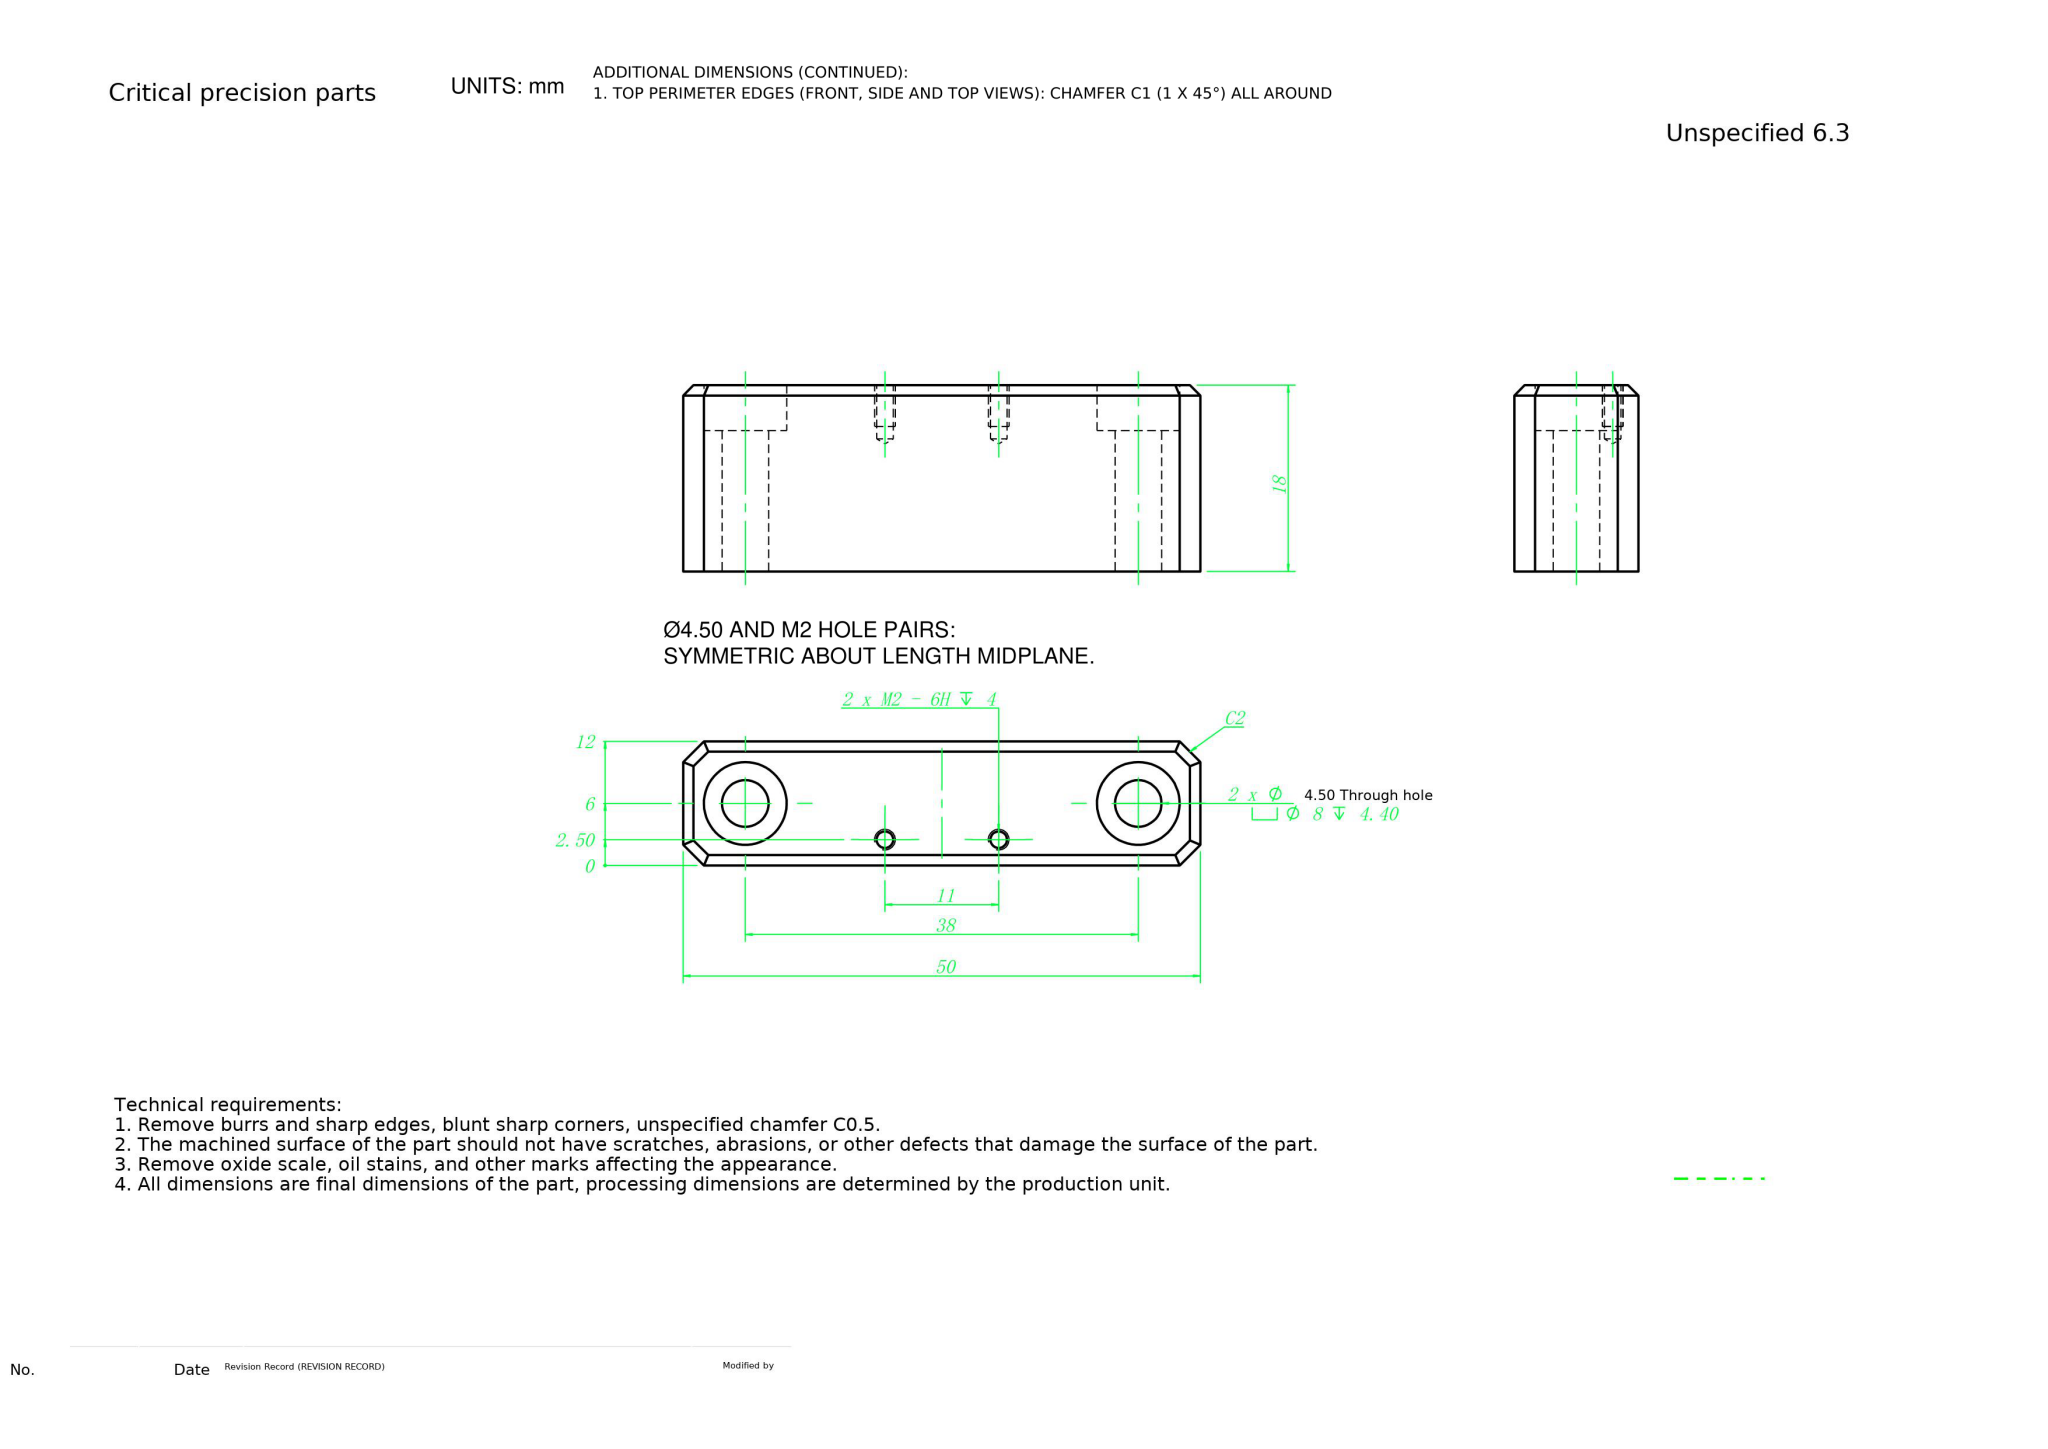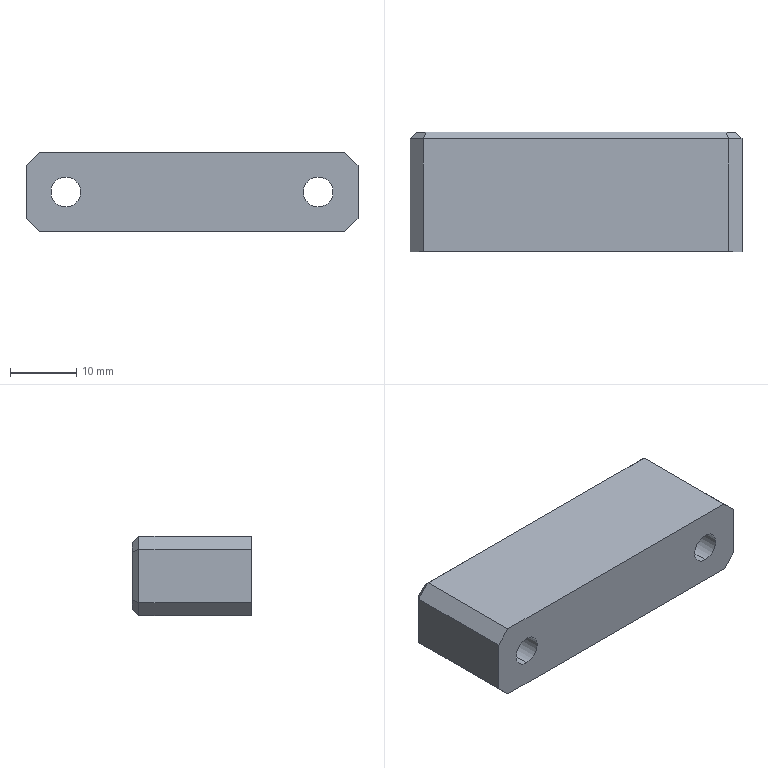Part | NX | mm | 1 solid | 36 faces | box 50 x 18 x 12 mm | volume 9701 mm3 | plane 20 | cylinder 12 | cone 4 | commonest cylinder face diameters 1.6 x4 8 x4 4.5 x4
STEP:
#1=COLOUR_RGB('',0.7922,0.8196,0.9333);
#2=FILL_AREA_STYLE_COLOUR('',#1);
#3=FILL_AREA_STYLE('',(#2));
#4=SURFACE_STYLE_FILL_AREA(#3);
#5=SURFACE_SIDE_STYLE('',(#4));
#6=SURFACE_STYLE_USAGE(.BOTH.,#5);
#7=PRESENTATION_STYLE_ASSIGNMENT((#6));
#8=CARTESIAN_POINT('',(5.5,3.8,-4.3));
#9=VERTEX_POINT('',#8);
#10=CARTESIAN_POINT('',(5.5,3.8,-2.7));
#11=VERTEX_POINT('',#10);
#12=CARTESIAN_POINT('',(5.5,3.8,-3.5));
#13=DIRECTION('',(0.,1.,0.));
#14=DIRECTION('',(0.,0.,1.));
#15=AXIS2_PLACEMENT_3D('',#12,#13,#14);
#16=CIRCLE('',#15,0.8);
#17=EDGE_CURVE('',#9,#11,#16,.T.);
#18=ORIENTED_EDGE('',*,*,#17,.F.);
#19=CARTESIAN_POINT('',(5.5,9.,-4.3));
#20=VERTEX_POINT('',#19);
#21=CARTESIAN_POINT('',(5.5,9.,-4.3));
#22=DIRECTION('',(0.,1.,0.));
#23=VECTOR('',#22,1000.);
#24=LINE('',#21,#23);
#25=EDGE_CURVE('',#9,#20,#24,.T.);
#26=ORIENTED_EDGE('',*,*,#25,.T.);
#27=CARTESIAN_POINT('',(5.5,9.,-2.7));
#28=VERTEX_POINT('',#27);
#29=CARTESIAN_POINT('',(5.5,9.,-3.5));
#30=DIRECTION('',(0.,1.,0.));
#31=DIRECTION('',(0.,0.,1.));
#32=AXIS2_PLACEMENT_3D('',#29,#30,#31);
#33=CIRCLE('',#32,0.8);
#34=EDGE_CURVE('',#20,#28,#33,.T.);
#35=ORIENTED_EDGE('',*,*,#34,.T.);
#36=CARTESIAN_POINT('',(5.5,9.,-2.7));
#37=DIRECTION('',(0.,1.,0.));
#38=VECTOR('',#37,1000.);
#39=LINE('',#36,#38);
#40=EDGE_CURVE('',#11,#28,#39,.T.);
#41=ORIENTED_EDGE('',*,*,#40,.F.);
#42=EDGE_LOOP('',(#18,#26,#35,#41));
#43=FACE_OUTER_BOUND('',#42,.T.);
#44=CARTESIAN_POINT('',(5.5,9.,-3.5));
#45=DIRECTION('',(0.,1.,0.));
#46=DIRECTION('',(0.,0.,1.));
#47=AXIS2_PLACEMENT_3D('',#44,#45,#46);
#48=CYLINDRICAL_SURFACE('',#47,0.8);
#49=ADVANCED_FACE('',(#43),#48,.F.);
#50=CARTESIAN_POINT('',(5.5,3.319,-3.5));
#51=VERTEX_POINT('',#50);
#52=CARTESIAN_POINT('',(5.5,3.8,-2.7));
#53=DIRECTION('',(0.,0.515,0.8572));
#54=VECTOR('',#53,1000.);
#55=LINE('',#52,#54);
#56=EDGE_CURVE('',#51,#11,#55,.T.);
#57=ORIENTED_EDGE('',*,*,#56,.F.);
#58=CARTESIAN_POINT('',(5.5,3.8,-4.3));
#59=DIRECTION('',(0.,0.515,-0.8572));
#60=VECTOR('',#59,1000.);
#61=LINE('',#58,#60);
#62=EDGE_CURVE('',#51,#9,#61,.T.);
#63=ORIENTED_EDGE('',*,*,#62,.T.);
#64=ORIENTED_EDGE('',*,*,#17,.T.);
#65=EDGE_LOOP('',(#57,#63,#64));
#66=FACE_OUTER_BOUND('',#65,.T.);
#67=CARTESIAN_POINT('',(5.5,3.8,-3.5));
#68=DIRECTION('',(0.,1.,0.));
#69=DIRECTION('',(0.,0.,1.));
#70=AXIS2_PLACEMENT_3D('',#67,#68,#69);
#71=CONICAL_SURFACE('',#70,0.8,1.03);
#72=ADVANCED_FACE('',(#66),#71,.F.);
#73=CARTESIAN_POINT('',(-5.5,3.8,-4.3));
#74=VERTEX_POINT('',#73);
#75=CARTESIAN_POINT('',(-5.5,3.8,-2.7));
#76=VERTEX_POINT('',#75);
#77=CARTESIAN_POINT('',(-5.5,3.8,-3.5));
#78=DIRECTION('',(0.,1.,0.));
#79=DIRECTION('',(0.,0.,1.));
#80=AXIS2_PLACEMENT_3D('',#77,#78,#79);
#81=CIRCLE('',#80,0.8);
#82=EDGE_CURVE('',#74,#76,#81,.T.);
#83=ORIENTED_EDGE('',*,*,#82,.F.);
#84=CARTESIAN_POINT('',(-5.5,9.,-4.3));
#85=VERTEX_POINT('',#84);
#86=CARTESIAN_POINT('',(-5.5,9.,-4.3));
#87=DIRECTION('',(0.,1.,0.));
#88=VECTOR('',#87,1000.);
#89=LINE('',#86,#88);
#90=EDGE_CURVE('',#74,#85,#89,.T.);
#91=ORIENTED_EDGE('',*,*,#90,.T.);
#92=CARTESIAN_POINT('',(-5.5,9.,-2.7));
#93=VERTEX_POINT('',#92);
#94=CARTESIAN_POINT('',(-5.5,9.,-3.5));
#95=DIRECTION('',(0.,1.,0.));
#96=DIRECTION('',(0.,0.,1.));
#97=AXIS2_PLACEMENT_3D('',#94,#95,#96);
#98=CIRCLE('',#97,0.8);
#99=EDGE_CURVE('',#85,#93,#98,.T.);
#100=ORIENTED_EDGE('',*,*,#99,.T.);
#101=CARTESIAN_POINT('',(-5.5,9.,-2.7));
#102=DIRECTION('',(0.,1.,0.));
#103=VECTOR('',#102,1000.);
#104=LINE('',#101,#103);
#105=EDGE_CURVE('',#76,#93,#104,.T.);
#106=ORIENTED_EDGE('',*,*,#105,.F.);
#107=EDGE_LOOP('',(#83,#91,#100,#106));
#108=FACE_OUTER_BOUND('',#107,.T.);
#109=CARTESIAN_POINT('',(-5.5,9.,-3.5));
#110=DIRECTION('',(0.,1.,0.));
#111=DIRECTION('',(0.,0.,1.));
#112=AXIS2_PLACEMENT_3D('',#109,#110,#111);
#113=CYLINDRICAL_SURFACE('',#112,0.8);
#114=ADVANCED_FACE('',(#108),#113,.F.);
#115=CARTESIAN_POINT('',(-5.5,3.319,-3.5));
#116=VERTEX_POINT('',#115);
#117=CARTESIAN_POINT('',(-5.5,3.8,-2.7));
#118=DIRECTION('',(0.,0.515,0.8572));
#119=VECTOR('',#118,1000.);
#120=LINE('',#117,#119);
#121=EDGE_CURVE('',#116,#76,#120,.T.);
#122=ORIENTED_EDGE('',*,*,#121,.F.);
#123=CARTESIAN_POINT('',(-5.5,3.8,-4.3));
#124=DIRECTION('',(0.,0.515,-0.8572));
#125=VECTOR('',#124,1000.);
#126=LINE('',#123,#125);
#127=EDGE_CURVE('',#116,#74,#126,.T.);
#128=ORIENTED_EDGE('',*,*,#127,.T.);
#129=ORIENTED_EDGE('',*,*,#82,.T.);
#130=EDGE_LOOP('',(#122,#128,#129));
#131=FACE_OUTER_BOUND('',#130,.T.);
#132=CARTESIAN_POINT('',(-5.5,3.8,-3.5));
#133=DIRECTION('',(0.,1.,0.));
#134=DIRECTION('',(0.,0.,1.));
#135=AXIS2_PLACEMENT_3D('',#132,#133,#134);
#136=CONICAL_SURFACE('',#135,0.8,1.03);
#137=ADVANCED_FACE('',(#131),#136,.F.);
#138=CARTESIAN_POINT('',(19.,4.6,-4.));
#139=VERTEX_POINT('',#138);
#140=CARTESIAN_POINT('',(19.,4.6,4.));
#141=VERTEX_POINT('',#140);
#142=CARTESIAN_POINT('',(19.,4.6,-0.));
#143=DIRECTION('',(0.,1.,0.));
#144=DIRECTION('',(0.,0.,1.));
#145=AXIS2_PLACEMENT_3D('',#142,#143,#144);
#146=CIRCLE('',#145,4.);
#147=EDGE_CURVE('',#139,#141,#146,.T.);
#148=ORIENTED_EDGE('',*,*,#147,.F.);
#149=CARTESIAN_POINT('',(19.,9.,-4.));
#150=VERTEX_POINT('',#149);
#151=CARTESIAN_POINT('',(19.,9.,-4.));
#152=DIRECTION('',(0.,1.,0.));
#153=VECTOR('',#152,1000.);
#154=LINE('',#151,#153);
#155=EDGE_CURVE('',#139,#150,#154,.T.);
#156=ORIENTED_EDGE('',*,*,#155,.T.);
#157=CARTESIAN_POINT('',(19.,9.,4.));
#158=VERTEX_POINT('',#157);
#159=CARTESIAN_POINT('',(19.,9.,-0.));
#160=DIRECTION('',(0.,1.,0.));
#161=DIRECTION('',(0.,0.,1.));
#162=AXIS2_PLACEMENT_3D('',#159,#160,#161);
#163=CIRCLE('',#162,4.);
#164=EDGE_CURVE('',#150,#158,#163,.T.);
#165=ORIENTED_EDGE('',*,*,#164,.T.);
#166=CARTESIAN_POINT('',(19.,9.,4.));
#167=DIRECTION('',(0.,1.,0.));
#168=VECTOR('',#167,1000.);
#169=LINE('',#166,#168);
#170=EDGE_CURVE('',#141,#158,#169,.T.);
#171=ORIENTED_EDGE('',*,*,#170,.F.);
#172=EDGE_LOOP('',(#148,#156,#165,#171));
#173=FACE_OUTER_BOUND('',#172,.T.);
#174=CARTESIAN_POINT('',(19.,9.,-0.));
#175=DIRECTION('',(0.,1.,0.));
#176=DIRECTION('',(0.,0.,1.));
#177=AXIS2_PLACEMENT_3D('',#174,#175,#176);
#178=CYLINDRICAL_SURFACE('',#177,4.);
#179=ADVANCED_FACE('',(#173),#178,.F.);
#180=CARTESIAN_POINT('',(19.,-9.,-2.25));
#181=VERTEX_POINT('',#180);
#182=CARTESIAN_POINT('',(19.,-9.,2.25));
#183=VERTEX_POINT('',#182);
#184=CARTESIAN_POINT('',(19.,-9.,-0.));
#185=DIRECTION('',(0.,1.,0.));
#186=DIRECTION('',(0.,0.,1.));
#187=AXIS2_PLACEMENT_3D('',#184,#185,#186);
#188=CIRCLE('',#187,2.25);
#189=EDGE_CURVE('',#181,#183,#188,.T.);
#190=ORIENTED_EDGE('',*,*,#189,.F.);
#191=CARTESIAN_POINT('',(19.,4.6,-2.25));
#192=VERTEX_POINT('',#191);
#193=CARTESIAN_POINT('',(19.,9.,-2.25));
#194=DIRECTION('',(0.,1.,0.));
#195=VECTOR('',#194,1000.);
#196=LINE('',#193,#195);
#197=EDGE_CURVE('',#181,#192,#196,.T.);
#198=ORIENTED_EDGE('',*,*,#197,.T.);
#199=CARTESIAN_POINT('',(19.,4.6,2.25));
#200=VERTEX_POINT('',#199);
#201=CARTESIAN_POINT('',(19.,4.6,-0.));
#202=DIRECTION('',(0.,1.,0.));
#203=DIRECTION('',(0.,0.,1.));
#204=AXIS2_PLACEMENT_3D('',#201,#202,#203);
#205=CIRCLE('',#204,2.25);
#206=EDGE_CURVE('',#192,#200,#205,.T.);
#207=ORIENTED_EDGE('',*,*,#206,.T.);
#208=CARTESIAN_POINT('',(19.,9.,2.25));
#209=DIRECTION('',(0.,1.,0.));
#210=VECTOR('',#209,1000.);
#211=LINE('',#208,#210);
#212=EDGE_CURVE('',#183,#200,#211,.T.);
#213=ORIENTED_EDGE('',*,*,#212,.F.);
#214=EDGE_LOOP('',(#190,#198,#207,#213));
#215=FACE_OUTER_BOUND('',#214,.T.);
#216=CARTESIAN_POINT('',(19.,9.,-0.));
#217=DIRECTION('',(0.,1.,0.));
#218=DIRECTION('',(0.,0.,1.));
#219=AXIS2_PLACEMENT_3D('',#216,#217,#218);
#220=CYLINDRICAL_SURFACE('',#219,2.25);
#221=ADVANCED_FACE('',(#215),#220,.F.);
#222=CARTESIAN_POINT('',(-19.,4.6,-4.));
#223=VERTEX_POINT('',#222);
#224=CARTESIAN_POINT('',(-19.,4.6,4.));
#225=VERTEX_POINT('',#224);
#226=CARTESIAN_POINT('',(-19.,4.6,0.));
#227=DIRECTION('',(0.,1.,0.));
#228=DIRECTION('',(0.,0.,1.));
#229=AXIS2_PLACEMENT_3D('',#226,#227,#228);
#230=CIRCLE('',#229,4.);
#231=EDGE_CURVE('',#223,#225,#230,.T.);
#232=ORIENTED_EDGE('',*,*,#231,.F.);
#233=CARTESIAN_POINT('',(-19.,9.,-4.));
#234=VERTEX_POINT('',#233);
#235=CARTESIAN_POINT('',(-19.,9.,-4.));
#236=DIRECTION('',(0.,1.,0.));
#237=VECTOR('',#236,1000.);
#238=LINE('',#235,#237);
#239=EDGE_CURVE('',#223,#234,#238,.T.);
#240=ORIENTED_EDGE('',*,*,#239,.T.);
#241=CARTESIAN_POINT('',(-19.,9.,4.));
#242=VERTEX_POINT('',#241);
#243=CARTESIAN_POINT('',(-19.,9.,0.));
#244=DIRECTION('',(0.,1.,0.));
#245=DIRECTION('',(0.,0.,1.));
#246=AXIS2_PLACEMENT_3D('',#243,#244,#245);
#247=CIRCLE('',#246,4.);
#248=EDGE_CURVE('',#234,#242,#247,.T.);
#249=ORIENTED_EDGE('',*,*,#248,.T.);
#250=CARTESIAN_POINT('',(-19.,9.,4.));
#251=DIRECTION('',(0.,1.,0.));
#252=VECTOR('',#251,1000.);
#253=LINE('',#250,#252);
#254=EDGE_CURVE('',#225,#242,#253,.T.);
#255=ORIENTED_EDGE('',*,*,#254,.F.);
#256=EDGE_LOOP('',(#232,#240,#249,#255));
#257=FACE_OUTER_BOUND('',#256,.T.);
#258=CARTESIAN_POINT('',(-19.,9.,0.));
#259=DIRECTION('',(0.,1.,0.));
#260=DIRECTION('',(0.,0.,1.));
#261=AXIS2_PLACEMENT_3D('',#258,#259,#260);
#262=CYLINDRICAL_SURFACE('',#261,4.);
#263=ADVANCED_FACE('',(#257),#262,.F.);
#264=CARTESIAN_POINT('',(-19.,-9.,-2.25));
#265=VERTEX_POINT('',#264);
#266=CARTESIAN_POINT('',(-19.,-9.,2.25));
#267=VERTEX_POINT('',#266);
#268=CARTESIAN_POINT('',(-19.,-9.,0.));
#269=DIRECTION('',(0.,1.,0.));
#270=DIRECTION('',(0.,0.,1.));
#271=AXIS2_PLACEMENT_3D('',#268,#269,#270);
#272=CIRCLE('',#271,2.25);
#273=EDGE_CURVE('',#265,#267,#272,.T.);
#274=ORIENTED_EDGE('',*,*,#273,.F.);
#275=CARTESIAN_POINT('',(-19.,4.6,-2.25));
#276=VERTEX_POINT('',#275);
#277=CARTESIAN_POINT('',(-19.,9.,-2.25));
#278=DIRECTION('',(0.,1.,0.));
#279=VECTOR('',#278,1000.);
#280=LINE('',#277,#279);
#281=EDGE_CURVE('',#265,#276,#280,.T.);
#282=ORIENTED_EDGE('',*,*,#281,.T.);
#283=CARTESIAN_POINT('',(-19.,4.6,2.25));
#284=VERTEX_POINT('',#283);
#285=CARTESIAN_POINT('',(-19.,4.6,0.));
#286=DIRECTION('',(0.,1.,0.));
#287=DIRECTION('',(0.,0.,1.));
#288=AXIS2_PLACEMENT_3D('',#285,#286,#287);
#289=CIRCLE('',#288,2.25);
#290=EDGE_CURVE('',#276,#284,#289,.T.);
#291=ORIENTED_EDGE('',*,*,#290,.T.);
#292=CARTESIAN_POINT('',(-19.,9.,2.25));
#293=DIRECTION('',(0.,1.,0.));
#294=VECTOR('',#293,1000.);
#295=LINE('',#292,#294);
#296=EDGE_CURVE('',#267,#284,#295,.T.);
#297=ORIENTED_EDGE('',*,*,#296,.F.);
#298=EDGE_LOOP('',(#274,#282,#291,#297));
#299=FACE_OUTER_BOUND('',#298,.T.);
#300=CARTESIAN_POINT('',(-19.,9.,0.));
#301=DIRECTION('',(0.,1.,0.));
#302=DIRECTION('',(0.,0.,1.));
#303=AXIS2_PLACEMENT_3D('',#300,#301,#302);
#304=CYLINDRICAL_SURFACE('',#303,2.25);
#305=ADVANCED_FACE('',(#299),#304,.F.);
#306=CARTESIAN_POINT('',(25.,-9.,-4.));
#307=VERTEX_POINT('',#306);
#308=CARTESIAN_POINT('',(25.,8.,-4.));
#309=VERTEX_POINT('',#308);
#310=CARTESIAN_POINT('',(25.,9.,-4.));
#311=DIRECTION('',(0.,1.,0.));
#312=VECTOR('',#311,1000.);
#313=LINE('',#310,#312);
#314=EDGE_CURVE('',#307,#309,#313,.T.);
#315=ORIENTED_EDGE('',*,*,#314,.T.);
#316=CARTESIAN_POINT('',(25.,8.,4.));
#317=VERTEX_POINT('',#316);
#318=CARTESIAN_POINT('',(25.,8.,6.));
#319=DIRECTION('',(0.,0.,1.));
#320=VECTOR('',#319,1000.);
#321=LINE('',#318,#320);
#322=EDGE_CURVE('',#309,#317,#321,.T.);
#323=ORIENTED_EDGE('',*,*,#322,.T.);
#324=CARTESIAN_POINT('',(25.,-9.,4.));
#325=VERTEX_POINT('',#324);
#326=CARTESIAN_POINT('',(25.,-9.,4.));
#327=DIRECTION('',(0.,-1.,0.));
#328=VECTOR('',#327,1000.);
#329=LINE('',#326,#328);
#330=EDGE_CURVE('',#317,#325,#329,.T.);
#331=ORIENTED_EDGE('',*,*,#330,.T.);
#332=CARTESIAN_POINT('',(25.,-9.,6.));
#333=DIRECTION('',(0.,0.,-1.));
#334=VECTOR('',#333,1000.);
#335=LINE('',#332,#334);
#336=EDGE_CURVE('',#325,#307,#335,.T.);
#337=ORIENTED_EDGE('',*,*,#336,.T.);
#338=EDGE_LOOP('',(#315,#323,#331,#337));
#339=FACE_OUTER_BOUND('',#338,.T.);
#340=CARTESIAN_POINT('',(25.,9.,6.));
#341=DIRECTION('',(-1.,0.,0.));
#342=DIRECTION('',(0.,0.,1.));
#343=AXIS2_PLACEMENT_3D('',#340,#341,#342);
#344=PLANE('',#343);
#345=ADVANCED_FACE('',(#339),#344,.F.);
#346=CARTESIAN_POINT('',(5.5,9.,-3.5));
#347=DIRECTION('',(0.,1.,0.));
#348=DIRECTION('',(0.,0.,1.));
#349=AXIS2_PLACEMENT_3D('',#346,#347,#348);
#350=CIRCLE('',#349,0.8);
#351=EDGE_CURVE('',#28,#20,#350,.T.);
#352=ORIENTED_EDGE('',*,*,#351,.F.);
#353=ORIENTED_EDGE('',*,*,#34,.F.);
#354=EDGE_LOOP('',(#352,#353));
#355=FACE_BOUND('',#354,.T.);
#356=CARTESIAN_POINT('',(-5.5,9.,-3.5));
#357=DIRECTION('',(0.,1.,0.));
#358=DIRECTION('',(0.,0.,1.));
#359=AXIS2_PLACEMENT_3D('',#356,#357,#358);
#360=CIRCLE('',#359,0.8);
#361=EDGE_CURVE('',#93,#85,#360,.T.);
#362=ORIENTED_EDGE('',*,*,#361,.F.);
#363=ORIENTED_EDGE('',*,*,#99,.F.);
#364=EDGE_LOOP('',(#362,#363));
#365=FACE_BOUND('',#364,.T.);
#366=CARTESIAN_POINT('',(19.,9.,-0.));
#367=DIRECTION('',(0.,1.,0.));
#368=DIRECTION('',(0.,0.,1.));
#369=AXIS2_PLACEMENT_3D('',#366,#367,#368);
#370=CIRCLE('',#369,4.);
#371=EDGE_CURVE('',#158,#150,#370,.T.);
#372=ORIENTED_EDGE('',*,*,#371,.F.);
#373=ORIENTED_EDGE('',*,*,#164,.F.);
#374=EDGE_LOOP('',(#372,#373));
#375=FACE_BOUND('',#374,.T.);
#376=CARTESIAN_POINT('',(-19.,9.,0.));
#377=DIRECTION('',(0.,1.,0.));
#378=DIRECTION('',(0.,0.,1.));
#379=AXIS2_PLACEMENT_3D('',#376,#377,#378);
#380=CIRCLE('',#379,4.);
#381=EDGE_CURVE('',#242,#234,#380,.T.);
#382=ORIENTED_EDGE('',*,*,#381,.F.);
#383=ORIENTED_EDGE('',*,*,#248,.F.);
#384=EDGE_LOOP('',(#382,#383));
#385=FACE_BOUND('',#384,.T.);
#386=CARTESIAN_POINT('',(22.586,9.,-5.));
#387=VERTEX_POINT('',#386);
#388=CARTESIAN_POINT('',(-22.586,9.,-5.));
#389=VERTEX_POINT('',#388);
#390=CARTESIAN_POINT('',(-25.,9.,-5.));
#391=DIRECTION('',(-1.,0.,0.));
#392=VECTOR('',#391,1000.);
#393=LINE('',#390,#392);
#394=EDGE_CURVE('',#387,#389,#393,.T.);
#395=ORIENTED_EDGE('',*,*,#394,.T.);
#396=CARTESIAN_POINT('',(-24.,9.,-3.586));
#397=VERTEX_POINT('',#396);
#398=CARTESIAN_POINT('',(-24.293,9.,-3.293));
#399=DIRECTION('',(-0.7071,0.,0.7071));
#400=VECTOR('',#399,1000.);
#401=LINE('',#398,#400);
#402=EDGE_CURVE('',#389,#397,#401,.T.);
#403=ORIENTED_EDGE('',*,*,#402,.T.);
#404=CARTESIAN_POINT('',(-24.,9.,3.586));
#405=VERTEX_POINT('',#404);
#406=CARTESIAN_POINT('',(-24.,9.,6.));
#407=DIRECTION('',(0.,0.,1.));
#408=VECTOR('',#407,1000.);
#409=LINE('',#406,#408);
#410=EDGE_CURVE('',#397,#405,#409,.T.);
#411=ORIENTED_EDGE('',*,*,#410,.T.);
#412=CARTESIAN_POINT('',(-22.586,9.,5.));
#413=VERTEX_POINT('',#412);
#414=CARTESIAN_POINT('',(-22.293,9.,5.293));
#415=DIRECTION('',(0.7071,0.,0.7071));
#416=VECTOR('',#415,1000.);
#417=LINE('',#414,#416);
#418=EDGE_CURVE('',#405,#413,#417,.T.);
#419=ORIENTED_EDGE('',*,*,#418,.T.);
#420=CARTESIAN_POINT('',(22.586,9.,5.));
#421=VERTEX_POINT('',#420);
#422=CARTESIAN_POINT('',(23.,9.,5.));
#423=DIRECTION('',(1.,0.,0.));
#424=VECTOR('',#423,1000.);
#425=LINE('',#422,#424);
#426=EDGE_CURVE('',#413,#421,#425,.T.);
#427=ORIENTED_EDGE('',*,*,#426,.T.);
#428=CARTESIAN_POINT('',(24.,9.,3.586));
#429=VERTEX_POINT('',#428);
#430=CARTESIAN_POINT('',(24.293,9.,3.293));
#431=DIRECTION('',(0.7071,0.,-0.7071));
#432=VECTOR('',#431,1000.);
#433=LINE('',#430,#432);
#434=EDGE_CURVE('',#421,#429,#433,.T.);
#435=ORIENTED_EDGE('',*,*,#434,.T.);
#436=CARTESIAN_POINT('',(24.,9.,-3.586));
#437=VERTEX_POINT('',#436);
#438=CARTESIAN_POINT('',(24.,9.,6.));
#439=DIRECTION('',(0.,0.,-1.));
#440=VECTOR('',#439,1000.);
#441=LINE('',#438,#440);
#442=EDGE_CURVE('',#429,#437,#441,.T.);
#443=ORIENTED_EDGE('',*,*,#442,.T.);
#444=CARTESIAN_POINT('',(22.293,9.,-5.293));
#445=DIRECTION('',(-0.7071,0.,-0.7071));
#446=VECTOR('',#445,1000.);
#447=LINE('',#444,#446);
#448=EDGE_CURVE('',#437,#387,#447,.T.);
#449=ORIENTED_EDGE('',*,*,#448,.T.);
#450=EDGE_LOOP('',(#395,#403,#411,#419,#427,#435,#443,#449));
#451=FACE_OUTER_BOUND('',#450,.T.);
#452=CARTESIAN_POINT('',(-25.,9.,6.));
#453=DIRECTION('',(0.,-1.,0.));
#454=DIRECTION('',(0.,0.,-1.));
#455=AXIS2_PLACEMENT_3D('',#452,#453,#454);
#456=PLANE('',#455);
#457=ADVANCED_FACE('',(#355,#365,#375,#385,#451),#456,.F.);
#458=CARTESIAN_POINT('',(-25.,-9.,4.));
#459=VERTEX_POINT('',#458);
#460=CARTESIAN_POINT('',(-25.,8.,4.));
#461=VERTEX_POINT('',#460);
#462=CARTESIAN_POINT('',(-25.,9.,4.));
#463=DIRECTION('',(-0.,1.,0.));
#464=VECTOR('',#463,1000.);
#465=LINE('',#462,#464);
#466=EDGE_CURVE('',#459,#461,#465,.T.);
#467=ORIENTED_EDGE('',*,*,#466,.T.);
#468=CARTESIAN_POINT('',(-25.,8.,-4.));
#469=VERTEX_POINT('',#468);
#470=CARTESIAN_POINT('',(-25.,8.,6.));
#471=DIRECTION('',(0.,0.,-1.));
#472=VECTOR('',#471,1000.);
#473=LINE('',#470,#472);
#474=EDGE_CURVE('',#461,#469,#473,.T.);
#475=ORIENTED_EDGE('',*,*,#474,.T.);
#476=CARTESIAN_POINT('',(-25.,-9.,-4.));
#477=VERTEX_POINT('',#476);
#478=CARTESIAN_POINT('',(-25.,9.,-4.));
#479=DIRECTION('',(0.,-1.,0.));
#480=VECTOR('',#479,1000.);
#481=LINE('',#478,#480);
#482=EDGE_CURVE('',#469,#477,#481,.T.);
#483=ORIENTED_EDGE('',*,*,#482,.T.);
#484=CARTESIAN_POINT('',(-25.,-9.,6.));
#485=DIRECTION('',(0.,0.,-1.));
#486=VECTOR('',#485,1000.);
#487=LINE('',#484,#486);
#488=EDGE_CURVE('',#459,#477,#487,.T.);
#489=ORIENTED_EDGE('',*,*,#488,.F.);
#490=EDGE_LOOP('',(#467,#475,#483,#489));
#491=FACE_OUTER_BOUND('',#490,.T.);
#492=CARTESIAN_POINT('',(-25.,9.,6.));
#493=DIRECTION('',(1.,0.,0.));
#494=DIRECTION('',(-0.,1.,0.));
#495=AXIS2_PLACEMENT_3D('',#492,#493,#494);
#496=PLANE('',#495);
#497=ADVANCED_FACE('',(#491),#496,.F.);
#498=CARTESIAN_POINT('',(19.,-9.,-0.));
#499=DIRECTION('',(0.,1.,0.));
#500=DIRECTION('',(0.,0.,1.));
#501=AXIS2_PLACEMENT_3D('',#498,#499,#500);
#502=CIRCLE('',#501,2.25);
#503=EDGE_CURVE('',#183,#181,#502,.T.);
#504=ORIENTED_EDGE('',*,*,#503,.T.);
#505=ORIENTED_EDGE('',*,*,#189,.T.);
#506=EDGE_LOOP('',(#504,#505));
#507=FACE_BOUND('',#506,.T.);
#508=CARTESIAN_POINT('',(-19.,-9.,0.));
#509=DIRECTION('',(0.,1.,0.));
#510=DIRECTION('',(0.,0.,1.));
#511=AXIS2_PLACEMENT_3D('',#508,#509,#510);
#512=CIRCLE('',#511,2.25);
#513=EDGE_CURVE('',#267,#265,#512,.T.);
#514=ORIENTED_EDGE('',*,*,#513,.T.);
#515=ORIENTED_EDGE('',*,*,#273,.T.);
#516=EDGE_LOOP('',(#514,#515));
#517=FACE_BOUND('',#516,.T.);
#518=CARTESIAN_POINT('',(-23.,-9.,6.));
#519=VERTEX_POINT('',#518);
#520=CARTESIAN_POINT('',(23.,-9.,6.));
#521=VERTEX_POINT('',#520);
#522=CARTESIAN_POINT('',(-25.,-9.,6.));
#523=DIRECTION('',(1.,0.,0.));
#524=VECTOR('',#523,1000.);
#525=LINE('',#522,#524);
#526=EDGE_CURVE('',#519,#521,#525,.T.);
#527=ORIENTED_EDGE('',*,*,#526,.F.);
#528=CARTESIAN_POINT('',(-23.,-9.,6.));
#529=DIRECTION('',(-0.7071,0.,-0.7071));
#530=VECTOR('',#529,1000.);
#531=LINE('',#528,#530);
#532=EDGE_CURVE('',#519,#459,#531,.T.);
#533=ORIENTED_EDGE('',*,*,#532,.T.);
#534=ORIENTED_EDGE('',*,*,#488,.T.);
#535=CARTESIAN_POINT('',(-23.,-9.,-6.));
#536=VERTEX_POINT('',#535);
#537=CARTESIAN_POINT('',(-25.,-9.,-4.));
#538=DIRECTION('',(0.7071,0.,-0.7071));
#539=VECTOR('',#538,1000.);
#540=LINE('',#537,#539);
#541=EDGE_CURVE('',#477,#536,#540,.T.);
#542=ORIENTED_EDGE('',*,*,#541,.T.);
#543=CARTESIAN_POINT('',(23.,-9.,-6.));
#544=VERTEX_POINT('',#543);
#545=CARTESIAN_POINT('',(-25.,-9.,-6.));
#546=DIRECTION('',(1.,0.,0.));
#547=VECTOR('',#546,1000.);
#548=LINE('',#545,#547);
#549=EDGE_CURVE('',#536,#544,#548,.T.);
#550=ORIENTED_EDGE('',*,*,#549,.T.);
#551=CARTESIAN_POINT('',(25.,-9.,-4.));
#552=DIRECTION('',(0.7071,0.,0.7071));
#553=VECTOR('',#552,1000.);
#554=LINE('',#551,#553);
#555=EDGE_CURVE('',#544,#307,#554,.T.);
#556=ORIENTED_EDGE('',*,*,#555,.T.);
#557=ORIENTED_EDGE('',*,*,#336,.F.);
#558=CARTESIAN_POINT('',(23.,-9.,6.));
#559=DIRECTION('',(-0.7071,0.,0.7071));
#560=VECTOR('',#559,1000.);
#561=LINE('',#558,#560);
#562=EDGE_CURVE('',#325,#521,#561,.T.);
#563=ORIENTED_EDGE('',*,*,#562,.T.);
#564=EDGE_LOOP('',(#527,#533,#534,#542,#550,#556,#557,#563));
#565=FACE_OUTER_BOUND('',#564,.T.);
#566=CARTESIAN_POINT('',(-25.,-9.,6.));
#567=DIRECTION('',(0.,1.,0.));
#568=DIRECTION('',(0.,0.,1.));
#569=AXIS2_PLACEMENT_3D('',#566,#567,#568);
#570=PLANE('',#569);
#571=ADVANCED_FACE('',(#507,#517,#565),#570,.F.);
#572=CARTESIAN_POINT('',(23.,8.,6.));
#573=VERTEX_POINT('',#572);
#574=CARTESIAN_POINT('',(23.,9.,6.));
#575=DIRECTION('',(0.,1.,0.));
#576=VECTOR('',#575,1000.);
#577=LINE('',#574,#576);
#578=EDGE_CURVE('',#521,#573,#577,.T.);
#579=ORIENTED_EDGE('',*,*,#578,.T.);
#580=CARTESIAN_POINT('',(-23.,8.,6.));
#581=VERTEX_POINT('',#580);
#582=CARTESIAN_POINT('',(-23.,8.,6.));
#583=DIRECTION('',(-1.,0.,0.));
#584=VECTOR('',#583,1000.);
#585=LINE('',#582,#584);
#586=EDGE_CURVE('',#573,#581,#585,.T.);
#587=ORIENTED_EDGE('',*,*,#586,.T.);
#588=CARTESIAN_POINT('',(-23.,-9.,6.));
#589=DIRECTION('',(0.,-1.,0.));
#590=VECTOR('',#589,1000.);
#591=LINE('',#588,#590);
#592=EDGE_CURVE('',#581,#519,#591,.T.);
#593=ORIENTED_EDGE('',*,*,#592,.T.);
#594=ORIENTED_EDGE('',*,*,#526,.T.);
#595=EDGE_LOOP('',(#579,#587,#593,#594));
#596=FACE_OUTER_BOUND('',#595,.T.);
#597=CARTESIAN_POINT('',(0.,0.,6.));
#598=DIRECTION('',(0.,0.,1.));
#599=DIRECTION('',(1.,0.,0.));
#600=AXIS2_PLACEMENT_3D('',#597,#598,#599);
#601=PLANE('',#600);
#602=ADVANCED_FACE('',(#596),#601,.T.);
#603=CARTESIAN_POINT('',(-23.,8.,-6.));
#604=VERTEX_POINT('',#603);
#605=CARTESIAN_POINT('',(-23.,-0.,-6.));
#606=DIRECTION('',(-0.,1.,0.));
#607=VECTOR('',#606,1000.);
#608=LINE('',#605,#607);
#609=EDGE_CURVE('',#536,#604,#608,.T.);
#610=ORIENTED_EDGE('',*,*,#609,.T.);
#611=CARTESIAN_POINT('',(23.,8.,-6.));
#612=VERTEX_POINT('',#611);
#613=CARTESIAN_POINT('',(0.,8.,-6.));
#614=DIRECTION('',(1.,0.,0.));
#615=VECTOR('',#614,1000.);
#616=LINE('',#613,#615);
#617=EDGE_CURVE('',#604,#612,#616,.T.);
#618=ORIENTED_EDGE('',*,*,#617,.T.);
#619=CARTESIAN_POINT('',(23.,0.,-6.));
#620=DIRECTION('',(0.,-1.,0.));
#621=VECTOR('',#620,1000.);
#622=LINE('',#619,#621);
#623=EDGE_CURVE('',#612,#544,#622,.T.);
#624=ORIENTED_EDGE('',*,*,#623,.T.);
#625=ORIENTED_EDGE('',*,*,#549,.F.);
#626=EDGE_LOOP('',(#610,#618,#624,#625));
#627=FACE_OUTER_BOUND('',#626,.T.);
#628=CARTESIAN_POINT('',(0.,0.,-6.));
#629=DIRECTION('',(0.,0.,1.));
#630=DIRECTION('',(1.,0.,0.));
#631=AXIS2_PLACEMENT_3D('',#628,#629,#630);
#632=PLANE('',#631);
#633=ADVANCED_FACE('',(#627),#632,.F.);
#634=ORIENTED_EDGE('',*,*,#592,.F.);
#635=CARTESIAN_POINT('',(-25.,8.,4.));
#636=DIRECTION('',(-0.7071,0.,-0.7071));
#637=VECTOR('',#636,1000.);
#638=LINE('',#635,#637);
#639=EDGE_CURVE('',#581,#461,#638,.T.);
#640=ORIENTED_EDGE('',*,*,#639,.T.);
#641=ORIENTED_EDGE('',*,*,#466,.F.);
#642=ORIENTED_EDGE('',*,*,#532,.F.);
#643=EDGE_LOOP('',(#634,#640,#641,#642));
#644=FACE_OUTER_BOUND('',#643,.T.);
#645=CARTESIAN_POINT('',(-23.,-0.,6.));
#646=DIRECTION('',(-0.7071,-0.,0.7071));
#647=DIRECTION('',(-0.,1.,0.));
#648=AXIS2_PLACEMENT_3D('',#645,#646,#647);
#649=PLANE('',#648);
#650=ADVANCED_FACE('',(#644),#649,.T.);
#651=ORIENTED_EDGE('',*,*,#330,.F.);
#652=CARTESIAN_POINT('',(23.,8.,6.));
#653=DIRECTION('',(-0.7071,0.,0.7071));
#654=VECTOR('',#653,1000.);
#655=LINE('',#652,#654);
#656=EDGE_CURVE('',#317,#573,#655,.T.);
#657=ORIENTED_EDGE('',*,*,#656,.T.);
#658=ORIENTED_EDGE('',*,*,#578,.F.);
#659=ORIENTED_EDGE('',*,*,#562,.F.);
#660=EDGE_LOOP('',(#651,#657,#658,#659));
#661=FACE_OUTER_BOUND('',#660,.T.);
#662=CARTESIAN_POINT('',(23.,0.,6.));
#663=DIRECTION('',(0.7071,0.,0.7071));
#664=DIRECTION('',(0.,-1.,0.));
#665=AXIS2_PLACEMENT_3D('',#662,#663,#664);
#666=PLANE('',#665);
#667=ADVANCED_FACE('',(#661),#666,.T.);
#668=ORIENTED_EDGE('',*,*,#482,.F.);
#669=CARTESIAN_POINT('',(-23.,8.,-6.));
#670=DIRECTION('',(0.7071,0.,-0.7071));
#671=VECTOR('',#670,1000.);
#672=LINE('',#669,#671);
#673=EDGE_CURVE('',#469,#604,#672,.T.);
#674=ORIENTED_EDGE('',*,*,#673,.T.);
#675=ORIENTED_EDGE('',*,*,#609,.F.);
#676=ORIENTED_EDGE('',*,*,#541,.F.);
#677=EDGE_LOOP('',(#668,#674,#675,#676));
#678=FACE_OUTER_BOUND('',#677,.T.);
#679=CARTESIAN_POINT('',(-25.,9.,-4.));
#680=DIRECTION('',(0.7071,0.,0.7071));
#681=DIRECTION('',(0.,-1.,0.));
#682=AXIS2_PLACEMENT_3D('',#679,#680,#681);
#683=PLANE('',#682);
#684=ADVANCED_FACE('',(#678),#683,.F.);
#685=ORIENTED_EDGE('',*,*,#623,.F.);
#686=CARTESIAN_POINT('',(25.,8.,-4.));
#687=DIRECTION('',(0.7071,0.,0.7071));
#688=VECTOR('',#687,1000.);
#689=LINE('',#686,#688);
#690=EDGE_CURVE('',#612,#309,#689,.T.);
#691=ORIENTED_EDGE('',*,*,#690,.T.);
#692=ORIENTED_EDGE('',*,*,#314,.F.);
#693=ORIENTED_EDGE('',*,*,#555,.F.);
#694=EDGE_LOOP('',(#685,#691,#692,#693));
#695=FACE_OUTER_BOUND('',#694,.T.);
#696=CARTESIAN_POINT('',(25.,9.,-4.));
#697=DIRECTION('',(-0.7071,0.,0.7071));
#698=DIRECTION('',(0.,1.,0.));
#699=AXIS2_PLACEMENT_3D('',#696,#697,#698);
#700=PLANE('',#699);
#701=ADVANCED_FACE('',(#695),#700,.F.);
#702=CARTESIAN_POINT('',(21.183,12.387,1.613));
#703=DIRECTION('',(-0.2811,0.6786,-0.6786));
#704=VECTOR('',#703,1000.);
#705=LINE('',#702,#704);
#706=EDGE_CURVE('',#573,#421,#705,.T.);
#707=ORIENTED_EDGE('',*,*,#706,.F.);
#708=ORIENTED_EDGE('',*,*,#656,.F.);
#709=CARTESIAN_POINT('',(17.065,15.935,0.7134));
#710=DIRECTION('',(0.6786,-0.6786,0.2811));
#711=VECTOR('',#710,1000.);
#712=LINE('',#709,#711);
#713=EDGE_CURVE('',#429,#317,#712,.T.);
#714=ORIENTED_EDGE('',*,*,#713,.F.);
#715=ORIENTED_EDGE('',*,*,#434,.F.);
#716=EDGE_LOOP('',(#707,#708,#714,#715));
#717=FACE_OUTER_BOUND('',#716,.T.);
#718=CARTESIAN_POINT('',(-1.707,9.,29.293));
#719=DIRECTION('',(0.5,0.7071,0.5));
#720=DIRECTION('',(-0.7071,0.,0.7071));
#721=AXIS2_PLACEMENT_3D('',#718,#719,#720);
#722=PLANE('',#721);
#723=ADVANCED_FACE('',(#717),#722,.T.);
#724=ORIENTED_EDGE('',*,*,#713,.T.);
#725=ORIENTED_EDGE('',*,*,#322,.F.);
#726=CARTESIAN_POINT('',(22.172,10.828,-2.828));
#727=DIRECTION('',(0.6786,-0.6786,-0.2811));
#728=VECTOR('',#727,1000.);
#729=LINE('',#726,#728);
#730=EDGE_CURVE('',#437,#309,#729,.T.);
#731=ORIENTED_EDGE('',*,*,#730,.F.);
#732=ORIENTED_EDGE('',*,*,#442,.F.);
#733=EDGE_LOOP('',(#724,#725,#731,#732));
#734=FACE_OUTER_BOUND('',#733,.T.);
#735=CARTESIAN_POINT('',(24.,9.,6.));
#736=DIRECTION('',(-0.7071,-0.7071,0.));
#737=DIRECTION('',(0.,0.,-1.));
#738=AXIS2_PLACEMENT_3D('',#735,#736,#737);
#739=PLANE('',#738);
#740=ADVANCED_FACE('',(#734),#739,.F.);
#741=ORIENTED_EDGE('',*,*,#706,.T.);
#742=ORIENTED_EDGE('',*,*,#426,.F.);
#743=CARTESIAN_POINT('',(-22.507,9.191,4.809));
#744=DIRECTION('',(0.2811,0.6786,-0.6786));
#745=VECTOR('',#744,1000.);
#746=LINE('',#743,#745);
#747=EDGE_CURVE('',#581,#413,#746,.T.);
#748=ORIENTED_EDGE('',*,*,#747,.F.);
#749=ORIENTED_EDGE('',*,*,#586,.F.);
#750=EDGE_LOOP('',(#741,#742,#748,#749));
#751=FACE_OUTER_BOUND('',#750,.T.);
#752=CARTESIAN_POINT('',(0.,8.,6.));
#753=DIRECTION('',(0.,0.7071,0.7071));
#754=DIRECTION('',(1.,0.,0.));
#755=AXIS2_PLACEMENT_3D('',#752,#753,#754);
#756=PLANE('',#755);
#757=ADVANCED_FACE('',(#751),#756,.T.);
#758=ORIENTED_EDGE('',*,*,#730,.T.);
#759=ORIENTED_EDGE('',*,*,#690,.F.);
#760=CARTESIAN_POINT('',(24.63,4.065,-9.935));
#761=DIRECTION('',(0.2811,-0.6786,-0.6786));
#762=VECTOR('',#761,1000.);
#763=LINE('',#760,#762);
#764=EDGE_CURVE('',#387,#612,#763,.T.);
#765=ORIENTED_EDGE('',*,*,#764,.F.);
#766=ORIENTED_EDGE('',*,*,#448,.F.);
#767=EDGE_LOOP('',(#758,#759,#765,#766));
#768=FACE_OUTER_BOUND('',#767,.T.);
#769=CARTESIAN_POINT('',(4.293,9.,-23.293));
#770=DIRECTION('',(-0.5,-0.7071,0.5));
#771=DIRECTION('',(-0.7071,0.,-0.7071));
#772=AXIS2_PLACEMENT_3D('',#769,#770,#771);
#773=PLANE('',#772);
#774=ADVANCED_FACE('',(#768),#773,.F.);
#775=ORIENTED_EDGE('',*,*,#747,.T.);
#776=ORIENTED_EDGE('',*,*,#418,.F.);
#777=CARTESIAN_POINT('',(-25.381,7.619,4.158));
#778=DIRECTION('',(0.6786,0.6786,-0.2811));
#779=VECTOR('',#778,1000.);
#780=LINE('',#777,#779);
#781=EDGE_CURVE('',#461,#405,#780,.T.);
#782=ORIENTED_EDGE('',*,*,#781,.F.);
#783=ORIENTED_EDGE('',*,*,#639,.F.);
#784=EDGE_LOOP('',(#775,#776,#782,#783));
#785=FACE_OUTER_BOUND('',#784,.T.);
#786=CARTESIAN_POINT('',(-23.293,9.,4.293));
#787=DIRECTION('',(-0.5,0.7071,0.5));
#788=DIRECTION('',(-0.7071,0.,-0.7071));
#789=AXIS2_PLACEMENT_3D('',#786,#787,#788);
#790=PLANE('',#789);
#791=ADVANCED_FACE('',(#785),#790,.T.);
#792=ORIENTED_EDGE('',*,*,#764,.T.);
#793=ORIENTED_EDGE('',*,*,#617,.F.);
#794=CARTESIAN_POINT('',(-22.777,8.54,-5.46));
#795=DIRECTION('',(-0.2811,-0.6786,-0.6786));
#796=VECTOR('',#795,1000.);
#797=LINE('',#794,#796);
#798=EDGE_CURVE('',#389,#604,#797,.T.);
#799=ORIENTED_EDGE('',*,*,#798,.F.);
#800=ORIENTED_EDGE('',*,*,#394,.F.);
#801=EDGE_LOOP('',(#792,#793,#799,#800));
#802=FACE_OUTER_BOUND('',#801,.T.);
#803=CARTESIAN_POINT('',(-25.,9.,-5.));
#804=DIRECTION('',(0.,-0.7071,0.7071));
#805=DIRECTION('',(-1.,0.,0.));
#806=AXIS2_PLACEMENT_3D('',#803,#804,#805);
#807=PLANE('',#806);
#808=ADVANCED_FACE('',(#802),#807,.F.);
#809=ORIENTED_EDGE('',*,*,#781,.T.);
#810=ORIENTED_EDGE('',*,*,#410,.F.);
#811=CARTESIAN_POINT('',(-23.093,9.907,-3.21));
#812=DIRECTION('',(0.6786,0.6786,0.2811));
#813=VECTOR('',#812,1000.);
#814=LINE('',#811,#813);
#815=EDGE_CURVE('',#469,#397,#814,.T.);
#816=ORIENTED_EDGE('',*,*,#815,.F.);
#817=ORIENTED_EDGE('',*,*,#474,.F.);
#818=EDGE_LOOP('',(#809,#810,#816,#817));
#819=FACE_OUTER_BOUND('',#818,.T.);
#820=CARTESIAN_POINT('',(-25.,8.,6.));
#821=DIRECTION('',(0.7071,-0.7071,0.));
#822=DIRECTION('',(0.,0.,-1.));
#823=AXIS2_PLACEMENT_3D('',#820,#821,#822);
#824=PLANE('',#823);
#825=ADVANCED_FACE('',(#819),#824,.F.);
#826=ORIENTED_EDGE('',*,*,#798,.T.);
#827=ORIENTED_EDGE('',*,*,#673,.F.);
#828=ORIENTED_EDGE('',*,*,#815,.T.);
#829=ORIENTED_EDGE('',*,*,#402,.F.);
#830=EDGE_LOOP('',(#826,#827,#828,#829));
#831=FACE_OUTER_BOUND('',#830,.T.);
#832=CARTESIAN_POINT('',(-29.293,9.,1.707));
#833=DIRECTION('',(0.5,-0.7071,0.5));
#834=DIRECTION('',(-0.7071,0.,0.7071));
#835=AXIS2_PLACEMENT_3D('',#832,#833,#834);
#836=PLANE('',#835);
#837=ADVANCED_FACE('',(#831),#836,.F.);
#838=ORIENTED_EDGE('',*,*,#281,.F.);
#839=ORIENTED_EDGE('',*,*,#513,.F.);
#840=ORIENTED_EDGE('',*,*,#296,.T.);
#841=CARTESIAN_POINT('',(-19.,4.6,0.));
#842=DIRECTION('',(0.,1.,0.));
#843=DIRECTION('',(0.,0.,1.));
#844=AXIS2_PLACEMENT_3D('',#841,#842,#843);
#845=CIRCLE('',#844,2.25);
#846=EDGE_CURVE('',#284,#276,#845,.T.);
#847=ORIENTED_EDGE('',*,*,#846,.T.);
#848=EDGE_LOOP('',(#838,#839,#840,#847));
#849=FACE_OUTER_BOUND('',#848,.T.);
#850=CARTESIAN_POINT('',(-19.,9.,0.));
#851=DIRECTION('',(0.,1.,0.));
#852=DIRECTION('',(0.,0.,1.));
#853=AXIS2_PLACEMENT_3D('',#850,#851,#852);
#854=CYLINDRICAL_SURFACE('',#853,2.25);
#855=ADVANCED_FACE('',(#849),#854,.F.);
#856=ORIENTED_EDGE('',*,*,#846,.F.);
#857=ORIENTED_EDGE('',*,*,#290,.F.);
#858=EDGE_LOOP('',(#856,#857));
#859=FACE_BOUND('',#858,.T.);
#860=CARTESIAN_POINT('',(-19.,4.6,0.));
#861=DIRECTION('',(0.,1.,0.));
#862=DIRECTION('',(0.,0.,1.));
#863=AXIS2_PLACEMENT_3D('',#860,#861,#862);
#864=CIRCLE('',#863,4.);
#865=EDGE_CURVE('',#225,#223,#864,.T.);
#866=ORIENTED_EDGE('',*,*,#865,.T.);
#867=ORIENTED_EDGE('',*,*,#231,.T.);
#868=EDGE_LOOP('',(#866,#867));
#869=FACE_OUTER_BOUND('',#868,.T.);
#870=CARTESIAN_POINT('',(-16.75,4.6,0.));
#871=DIRECTION('',(0.,-1.,0.));
#872=DIRECTION('',(0.,0.,-1.));
#873=AXIS2_PLACEMENT_3D('',#870,#871,#872);
#874=PLANE('',#873);
#875=ADVANCED_FACE('',(#859,#869),#874,.F.);
#876=ORIENTED_EDGE('',*,*,#239,.F.);
#877=ORIENTED_EDGE('',*,*,#865,.F.);
#878=ORIENTED_EDGE('',*,*,#254,.T.);
#879=ORIENTED_EDGE('',*,*,#381,.T.);
#880=EDGE_LOOP('',(#876,#877,#878,#879));
#881=FACE_OUTER_BOUND('',#880,.T.);
#882=CARTESIAN_POINT('',(-19.,9.,0.));
#883=DIRECTION('',(0.,1.,0.));
#884=DIRECTION('',(0.,0.,1.));
#885=AXIS2_PLACEMENT_3D('',#882,#883,#884);
#886=CYLINDRICAL_SURFACE('',#885,4.);
#887=ADVANCED_FACE('',(#881),#886,.F.);
#888=ORIENTED_EDGE('',*,*,#197,.F.);
#889=ORIENTED_EDGE('',*,*,#503,.F.);
#890=ORIENTED_EDGE('',*,*,#212,.T.);
#891=CARTESIAN_POINT('',(19.,4.6,-0.));
#892=DIRECTION('',(0.,1.,0.));
#893=DIRECTION('',(0.,0.,1.));
#894=AXIS2_PLACEMENT_3D('',#891,#892,#893);
#895=CIRCLE('',#894,2.25);
#896=EDGE_CURVE('',#200,#192,#895,.T.);
#897=ORIENTED_EDGE('',*,*,#896,.T.);
#898=EDGE_LOOP('',(#888,#889,#890,#897));
#899=FACE_OUTER_BOUND('',#898,.T.);
#900=CARTESIAN_POINT('',(19.,9.,-0.));
#901=DIRECTION('',(0.,1.,0.));
#902=DIRECTION('',(0.,0.,1.));
#903=AXIS2_PLACEMENT_3D('',#900,#901,#902);
#904=CYLINDRICAL_SURFACE('',#903,2.25);
#905=ADVANCED_FACE('',(#899),#904,.F.);
#906=ORIENTED_EDGE('',*,*,#896,.F.);
#907=ORIENTED_EDGE('',*,*,#206,.F.);
#908=EDGE_LOOP('',(#906,#907));
#909=FACE_BOUND('',#908,.T.);
#910=CARTESIAN_POINT('',(19.,4.6,-0.));
#911=DIRECTION('',(0.,1.,0.));
#912=DIRECTION('',(0.,0.,1.));
#913=AXIS2_PLACEMENT_3D('',#910,#911,#912);
#914=CIRCLE('',#913,4.);
#915=EDGE_CURVE('',#141,#139,#914,.T.);
#916=ORIENTED_EDGE('',*,*,#915,.T.);
#917=ORIENTED_EDGE('',*,*,#147,.T.);
#918=EDGE_LOOP('',(#916,#917));
#919=FACE_OUTER_BOUND('',#918,.T.);
#920=CARTESIAN_POINT('',(21.25,4.6,-0.));
#921=DIRECTION('',(0.,-1.,0.));
#922=DIRECTION('',(0.,0.,-1.));
#923=AXIS2_PLACEMENT_3D('',#920,#921,#922);
#924=PLANE('',#923);
#925=ADVANCED_FACE('',(#909,#919),#924,.F.);
#926=ORIENTED_EDGE('',*,*,#155,.F.);
#927=ORIENTED_EDGE('',*,*,#915,.F.);
#928=ORIENTED_EDGE('',*,*,#170,.T.);
#929=ORIENTED_EDGE('',*,*,#371,.T.);
#930=EDGE_LOOP('',(#926,#927,#928,#929));
#931=FACE_OUTER_BOUND('',#930,.T.);
#932=CARTESIAN_POINT('',(19.,9.,-0.));
#933=DIRECTION('',(0.,1.,0.));
#934=DIRECTION('',(0.,0.,1.));
#935=AXIS2_PLACEMENT_3D('',#932,#933,#934);
#936=CYLINDRICAL_SURFACE('',#935,4.);
#937=ADVANCED_FACE('',(#931),#936,.F.);
#938=ORIENTED_EDGE('',*,*,#127,.F.);
#939=ORIENTED_EDGE('',*,*,#121,.T.);
#940=CARTESIAN_POINT('',(-5.5,3.8,-3.5));
#941=DIRECTION('',(0.,1.,0.));
#942=DIRECTION('',(0.,0.,1.));
#943=AXIS2_PLACEMENT_3D('',#940,#941,#942);
#944=CIRCLE('',#943,0.8);
#945=EDGE_CURVE('',#76,#74,#944,.T.);
#946=ORIENTED_EDGE('',*,*,#945,.T.);
#947=EDGE_LOOP('',(#938,#939,#946));
#948=FACE_OUTER_BOUND('',#947,.T.);
#949=CARTESIAN_POINT('',(-5.5,3.8,-3.5));
#950=DIRECTION('',(0.,1.,0.));
#951=DIRECTION('',(0.,0.,1.));
#952=AXIS2_PLACEMENT_3D('',#949,#950,#951);
#953=CONICAL_SURFACE('',#952,0.8,1.03);
#954=ADVANCED_FACE('',(#948),#953,.F.);
#955=ORIENTED_EDGE('',*,*,#90,.F.);
#956=ORIENTED_EDGE('',*,*,#945,.F.);
#957=ORIENTED_EDGE('',*,*,#105,.T.);
#958=ORIENTED_EDGE('',*,*,#361,.T.);
#959=EDGE_LOOP('',(#955,#956,#957,#958));
#960=FACE_OUTER_BOUND('',#959,.T.);
#961=CARTESIAN_POINT('',(-5.5,9.,-3.5));
#962=DIRECTION('',(0.,1.,0.));
#963=DIRECTION('',(0.,0.,1.));
#964=AXIS2_PLACEMENT_3D('',#961,#962,#963);
#965=CYLINDRICAL_SURFACE('',#964,0.8);
#966=ADVANCED_FACE('',(#960),#965,.F.);
#967=ORIENTED_EDGE('',*,*,#62,.F.);
#968=ORIENTED_EDGE('',*,*,#56,.T.);
#969=CARTESIAN_POINT('',(5.5,3.8,-3.5));
#970=DIRECTION('',(0.,1.,0.));
#971=DIRECTION('',(0.,0.,1.));
#972=AXIS2_PLACEMENT_3D('',#969,#970,#971);
#973=CIRCLE('',#972,0.8);
#974=EDGE_CURVE('',#11,#9,#973,.T.);
#975=ORIENTED_EDGE('',*,*,#974,.T.);
#976=EDGE_LOOP('',(#967,#968,#975));
#977=FACE_OUTER_BOUND('',#976,.T.);
#978=CARTESIAN_POINT('',(5.5,3.8,-3.5));
#979=DIRECTION('',(0.,1.,0.));
#980=DIRECTION('',(0.,0.,1.));
#981=AXIS2_PLACEMENT_3D('',#978,#979,#980);
#982=CONICAL_SURFACE('',#981,0.8,1.03);
#983=ADVANCED_FACE('',(#977),#982,.F.);
#984=ORIENTED_EDGE('',*,*,#25,.F.);
#985=ORIENTED_EDGE('',*,*,#974,.F.);
#986=ORIENTED_EDGE('',*,*,#40,.T.);
#987=ORIENTED_EDGE('',*,*,#351,.T.);
#988=EDGE_LOOP('',(#984,#985,#986,#987));
#989=FACE_OUTER_BOUND('',#988,.T.);
#990=CARTESIAN_POINT('',(5.5,9.,-3.5));
#991=DIRECTION('',(0.,1.,0.));
#992=DIRECTION('',(0.,0.,1.));
#993=AXIS2_PLACEMENT_3D('',#990,#991,#992);
#994=CYLINDRICAL_SURFACE('',#993,0.8);
#995=ADVANCED_FACE('',(#989),#994,.F.);
#996=CLOSED_SHELL('',(#49,#72,#114,#137,#179,#221,#263,#305,#345,#457,#497,#571,#602,#633,#650,#667,#684,#701,#723,#740,#757,#774,#791,#808,#825,#837,#855,#875,#887,#905,#925,#937,#954,#966,#983,#995));
#997=MANIFOLD_SOLID_BREP('',#996);
#998=STYLED_ITEM('',(#7),#997);
#999=PRESENTATION_LAYER_ASSIGNMENT('','',(#998));
#1000=(LENGTH_UNIT()NAMED_UNIT(*)SI_UNIT(.MILLI.,.METRE.));
#1001=UNCERTAINTY_MEASURE_WITH_UNIT(LENGTH_MEASURE(0.00001),#1000,'','');
#1002=(NAMED_UNIT(*)PLANE_ANGLE_UNIT()SI_UNIT($,.RADIAN.));
#1003=(NAMED_UNIT(*)SI_UNIT($,.STERADIAN.)SOLID_ANGLE_UNIT());
#1004=(GEOMETRIC_REPRESENTATION_CONTEXT(3)GLOBAL_UNCERTAINTY_ASSIGNED_CONTEXT((#1001))GLOBAL_UNIT_ASSIGNED_CONTEXT((#1000,#1002,#1003))REPRESENTATION_CONTEXT('',''));
#1005=MECHANICAL_DESIGN_GEOMETRIC_PRESENTATION_REPRESENTATION('',(#998),#1004);
#1006=CARTESIAN_POINT('',(0.,0.,0.));
#1007=DIRECTION('',(0.,0.,1.));
#1008=DIRECTION('',(1.,0.,0.));
#1009=AXIS2_PLACEMENT_3D('',#1006,#1007,#1008);
#1010=(LENGTH_UNIT()NAMED_UNIT(*)SI_UNIT(.MILLI.,.METRE.));
#1011=UNCERTAINTY_MEASURE_WITH_UNIT(LENGTH_MEASURE(0.00001),#1010,'','');
#1012=(NAMED_UNIT(*)PLANE_ANGLE_UNIT()SI_UNIT($,.RADIAN.));
#1013=(NAMED_UNIT(*)SI_UNIT($,.STERADIAN.)SOLID_ANGLE_UNIT());
#1014=(GEOMETRIC_REPRESENTATION_CONTEXT(3)GLOBAL_UNCERTAINTY_ASSIGNED_CONTEXT((#1011))GLOBAL_UNIT_ASSIGNED_CONTEXT((#1010,#1012,#1013))REPRESENTATION_CONTEXT('',''));
#1015=ADVANCED_BREP_SHAPE_REPRESENTATION('',(#997,#1009),#1014);